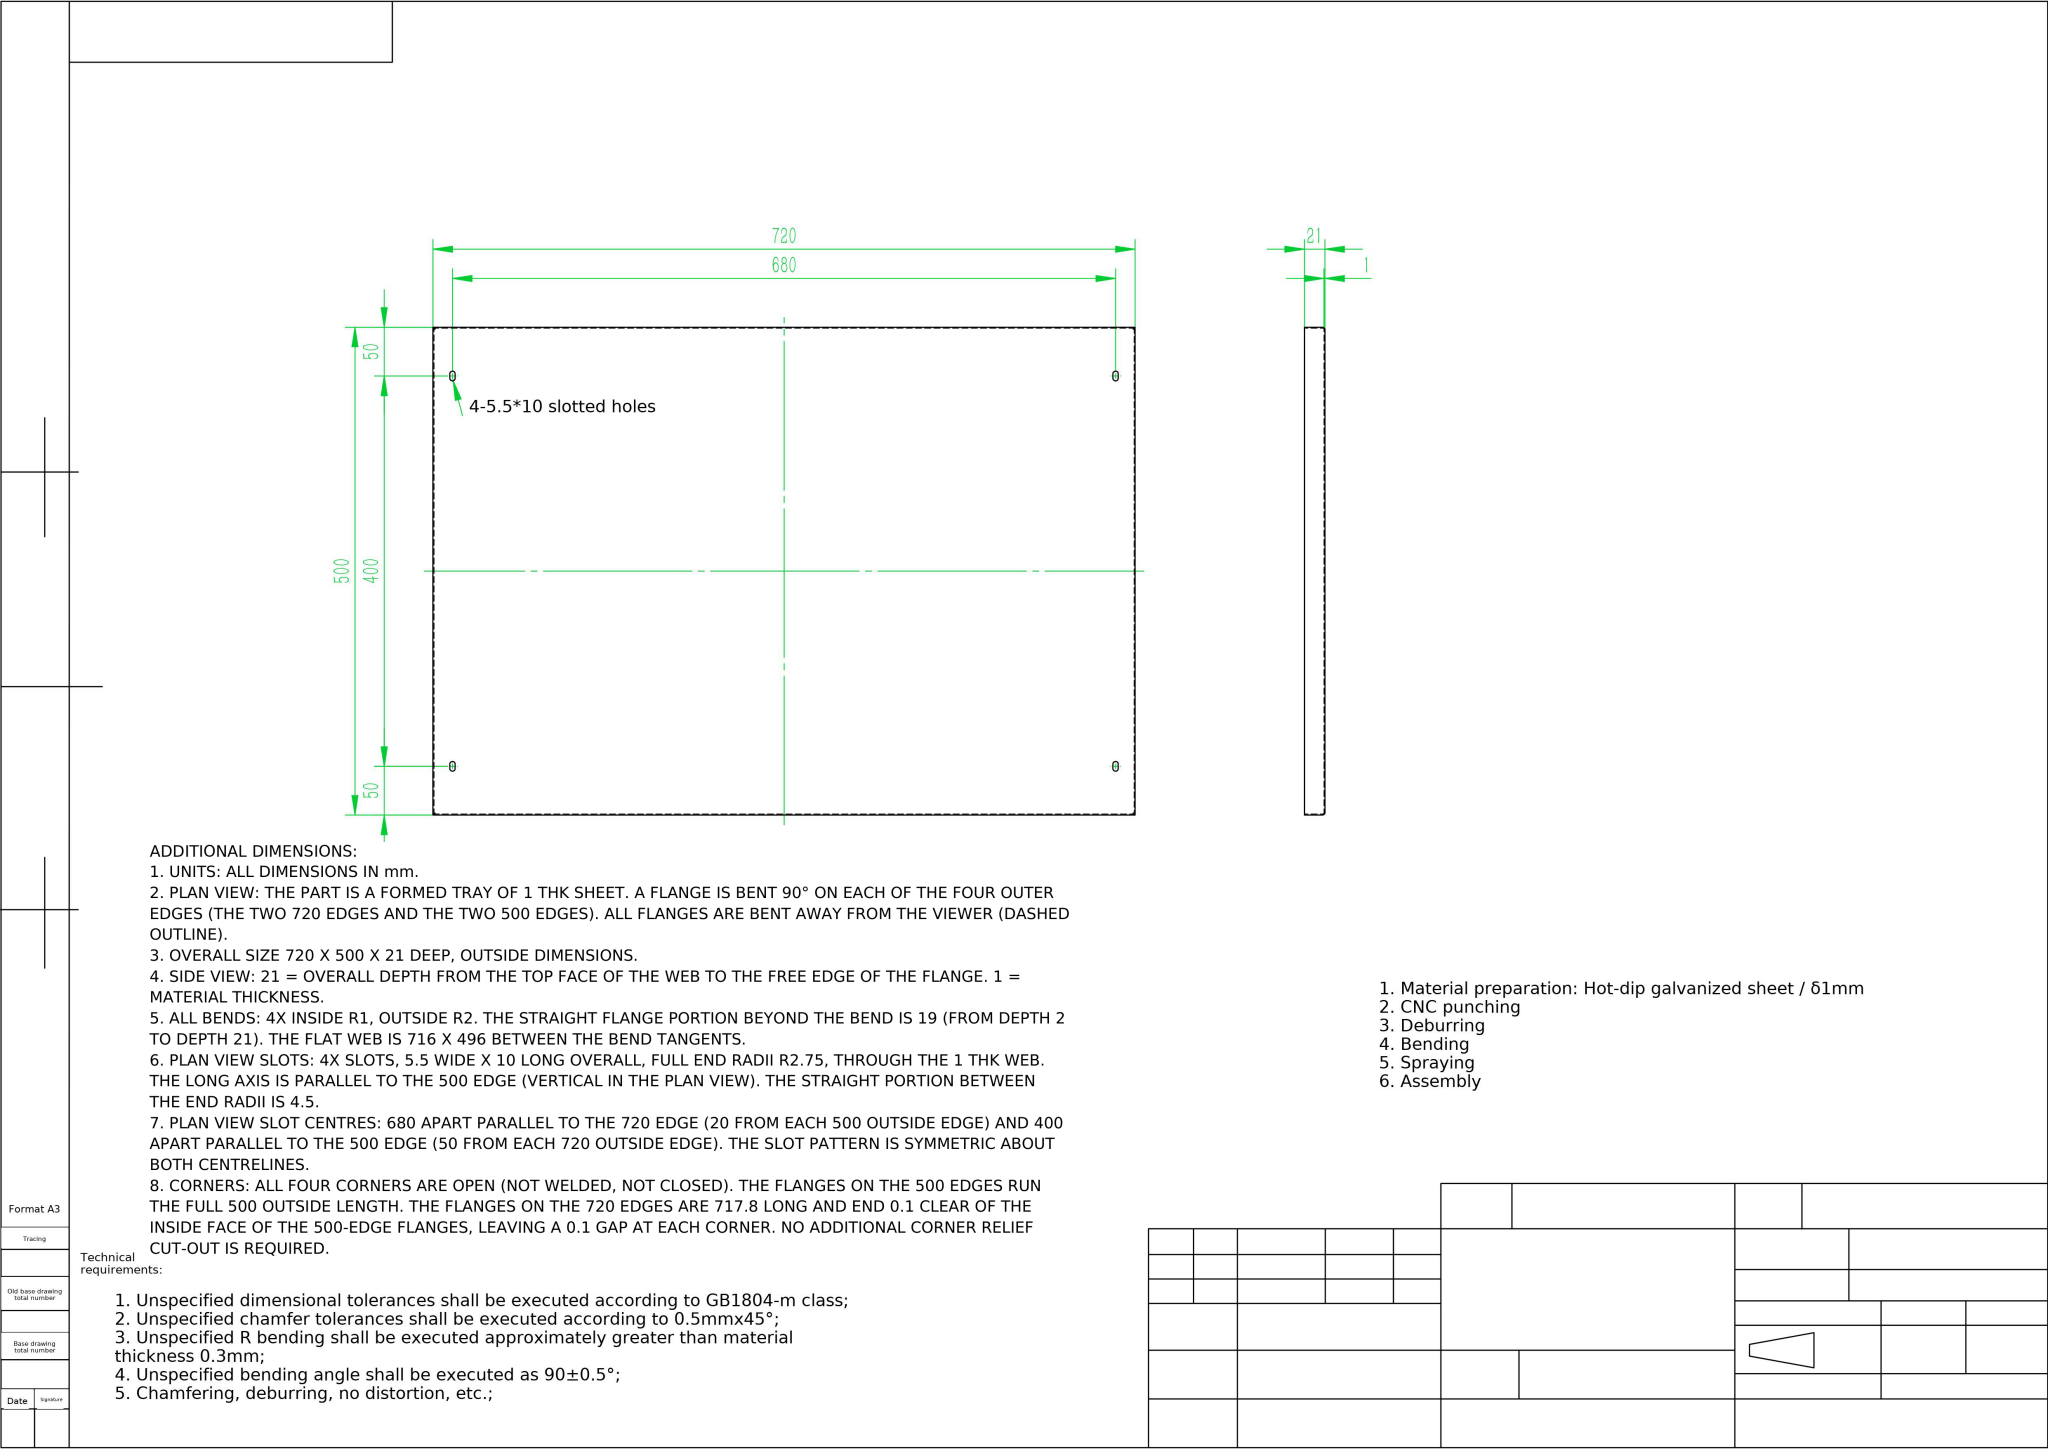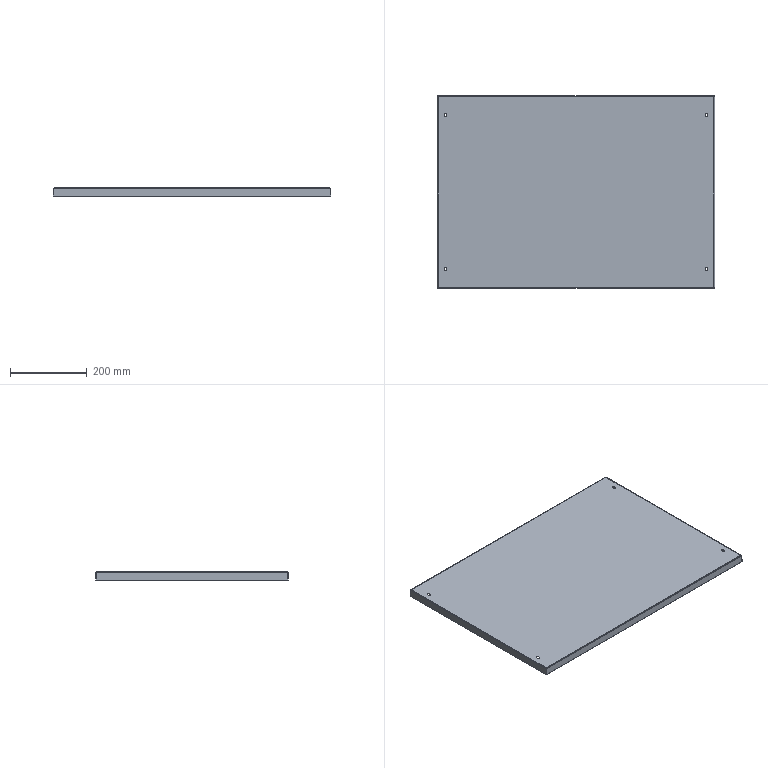Part | NX | mm | 1 solid | 54 faces | box 720 x 500 x 21 mm | volume 406943 mm3 | plane 30 | cylinder 16 | spline 8 | commonest cylinder face diameters 5.5 x8 2 x4 4 x4